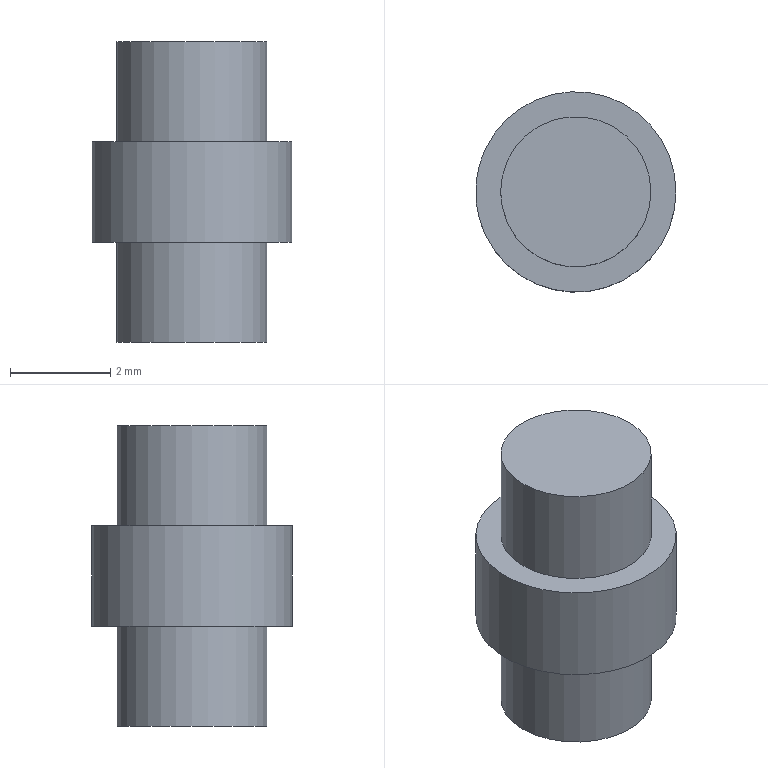Component | NX | CIRCUIT_PIN_2 | 1 solid | 7 faces | box 4 x 4 x 6 mm | volume 53 mm3 | plane 4 | cylinder 3 | commonest cylinder face diameters 3 x2 4 x1
STEP:
#1=CARTESIAN_POINT('',(0.,0.,0.));
#2=DIRECTION('',(0.,0.,1.));
#3=DIRECTION('',(1.,0.,0.));
#4=AXIS2_PLACEMENT_3D('',#1,#2,#3);
#5=CARTESIAN_POINT('',(22.205,25.006,-22.892));
#6=VERTEX_POINT('',#5);
#7=CARTESIAN_POINT('',(20.705,25.006,-22.892));
#8=DIRECTION('',(0.,0.,-1.));
#9=DIRECTION('',(1.,0.,0.));
#10=AXIS2_PLACEMENT_3D('',#7,#8,#9);
#11=CIRCLE('',#10,1.5);
#12=CARTESIAN_POINT('',(20.705,25.006,-22.892));
#13=DIRECTION('',(0.,0.,1.));
#14=DIRECTION('',(0.,-1.,0.));
#15=AXIS2_PLACEMENT_3D('',#12,#13,#14);
#16=PLANE('',#15);
#17=CARTESIAN_POINT('',(0.,1.5));
#18=CARTESIAN_POINT('',(2.598,1.5));
#19=CARTESIAN_POINT('',(1.299,-0.75));
#20=CARTESIAN_POINT('',(0.,-3.));
#21=CARTESIAN_POINT('',(-1.299,-0.75));
#22=CARTESIAN_POINT('',(-2.598,1.5));
#23=CARTESIAN_POINT('',(0.,1.5));
#24=(BOUNDED_CURVE()B_SPLINE_CURVE(2,(#17,#18,#19,#20,#21,#22,#23),.UNSPECIFIED.,.T.,.F.)B_SPLINE_CURVE_WITH_KNOTS((1,2,2,2,2,1),(-2.094,0.,2.094,4.189,6.283,8.378),.UNSPECIFIED.)CURVE()GEOMETRIC_REPRESENTATION_ITEM()RATIONAL_B_SPLINE_CURVE((1.,0.5,1.,0.5,1.,0.5,1.))REPRESENTATION_ITEM(''));
#25=(GEOMETRIC_REPRESENTATION_CONTEXT(2)PARAMETRIC_REPRESENTATION_CONTEXT()REPRESENTATION_CONTEXT('',''));
#26=DEFINITIONAL_REPRESENTATION('',(#24),#25);
#27=PCURVE('',#16,#26);
#28=CARTESIAN_POINT('',(20.705,25.006,-24.892));
#29=DIRECTION('',(0.,0.,1.));
#30=DIRECTION('',(1.,0.,0.));
#31=AXIS2_PLACEMENT_3D('',#28,#29,#30);
#32=CYLINDRICAL_SURFACE('',#31,1.5);
#33=CARTESIAN_POINT('',(6.283,2.));
#34=DIRECTION('',(-1.,0.));
#35=VECTOR('',#34,1.);
#36=LINE('',#33,#35);
#37=(GEOMETRIC_REPRESENTATION_CONTEXT(2)PARAMETRIC_REPRESENTATION_CONTEXT()REPRESENTATION_CONTEXT('',''));
#38=DEFINITIONAL_REPRESENTATION('',(#36),#37);
#39=PCURVE('',#32,#38);
#40=SURFACE_CURVE('',#11,(#27,#39),.PCURVE_S1.);
#41=EDGE_CURVE('',#6,#6,#40,.T.);
#42=ORIENTED_EDGE('',*,*,#41,.F.);
#43=EDGE_LOOP('',(#42));
#44=FACE_BOUND('',#43,.T.);
#45=ADVANCED_FACE('',(#44),#16,.T.);
#46=ORIENTED_EDGE('',*,*,#41,.T.);
#47=CARTESIAN_POINT('',(22.205,25.006,-24.892));
#48=VERTEX_POINT('',#47);
#49=CARTESIAN_POINT('',(22.205,25.006,-24.892));
#50=CARTESIAN_POINT('',(22.205,25.006,-22.892));
#51=B_SPLINE_CURVE_WITH_KNOTS('',1,(#49,#50),.UNSPECIFIED.,.F.,.F.,(2,2),(0.,2.),.PIECEWISE_BEZIER_KNOTS.);
#52=CARTESIAN_POINT('',(0.,0.));
#53=DIRECTION('',(0.,1.));
#54=VECTOR('',#53,1.);
#55=LINE('',#52,#54);
#56=(GEOMETRIC_REPRESENTATION_CONTEXT(2)PARAMETRIC_REPRESENTATION_CONTEXT()REPRESENTATION_CONTEXT('',''));
#57=DEFINITIONAL_REPRESENTATION('',(#55),#56);
#58=PCURVE('',#32,#57);
#59=CARTESIAN_POINT('',(6.283,0.));
#60=DIRECTION('',(0.,1.));
#61=VECTOR('',#60,1.);
#62=LINE('',#59,#61);
#63=(GEOMETRIC_REPRESENTATION_CONTEXT(2)PARAMETRIC_REPRESENTATION_CONTEXT()REPRESENTATION_CONTEXT('',''));
#64=DEFINITIONAL_REPRESENTATION('',(#62),#63);
#65=PCURVE('',#32,#64);
#66=SEAM_CURVE('',#51,(#58,#65),.PCURVE_S1.);
#67=EDGE_CURVE('',#48,#6,#66,.T.);
#68=ORIENTED_EDGE('',*,*,#67,.F.);
#69=CARTESIAN_POINT('',(20.705,25.006,-24.892));
#70=DIRECTION('',(0.,0.,1.));
#71=DIRECTION('',(1.,0.,0.));
#72=AXIS2_PLACEMENT_3D('',#69,#70,#71);
#73=CIRCLE('',#72,1.5);
#74=CARTESIAN_POINT('',(0.,0.));
#75=DIRECTION('',(1.,0.));
#76=VECTOR('',#75,1.);
#77=LINE('',#74,#76);
#78=(GEOMETRIC_REPRESENTATION_CONTEXT(2)PARAMETRIC_REPRESENTATION_CONTEXT()REPRESENTATION_CONTEXT('',''));
#79=DEFINITIONAL_REPRESENTATION('',(#77),#78);
#80=PCURVE('',#32,#79);
#81=CARTESIAN_POINT('',(20.705,25.006,-24.892));
#82=DIRECTION('',(0.,0.,1.));
#83=DIRECTION('',(0.,-1.,0.));
#84=AXIS2_PLACEMENT_3D('',#81,#82,#83);
#85=PLANE('',#84);
#86=CARTESIAN_POINT('',(0.,0.));
#87=DIRECTION('',(0.,1.));
#88=AXIS2_PLACEMENT_2D('',#86,#87);
#89=CIRCLE('',#88,1.5);
#90=(GEOMETRIC_REPRESENTATION_CONTEXT(2)PARAMETRIC_REPRESENTATION_CONTEXT()REPRESENTATION_CONTEXT('',''));
#91=DEFINITIONAL_REPRESENTATION('',(#89),#90);
#92=PCURVE('',#85,#91);
#93=SURFACE_CURVE('',#73,(#80,#92),.PCURVE_S1.);
#94=EDGE_CURVE('',#48,#48,#93,.T.);
#95=ORIENTED_EDGE('',*,*,#94,.T.);
#96=ORIENTED_EDGE('',*,*,#67,.T.);
#97=EDGE_LOOP('',(#46,#68,#95,#96));
#98=FACE_BOUND('',#97,.T.);
#99=ADVANCED_FACE('',(#98),#32,.T.);
#100=CARTESIAN_POINT('',(22.205,25.006,-26.892));
#101=VERTEX_POINT('',#100);
#102=CARTESIAN_POINT('',(20.705,25.006,-26.892));
#103=DIRECTION('',(0.,0.,-1.));
#104=DIRECTION('',(1.,0.,0.));
#105=AXIS2_PLACEMENT_3D('',#102,#103,#104);
#106=CIRCLE('',#105,1.5);
#107=CARTESIAN_POINT('',(20.705,25.006,-26.892));
#108=DIRECTION('',(0.,0.,-1.));
#109=DIRECTION('',(0.,1.,0.));
#110=AXIS2_PLACEMENT_3D('',#107,#108,#109);
#111=PLANE('',#110);
#112=CARTESIAN_POINT('',(0.,0.));
#113=DIRECTION('',(0.,1.));
#114=AXIS2_PLACEMENT_2D('',#112,#113);
#115=CIRCLE('',#114,1.5);
#116=(GEOMETRIC_REPRESENTATION_CONTEXT(2)PARAMETRIC_REPRESENTATION_CONTEXT()REPRESENTATION_CONTEXT('',''));
#117=DEFINITIONAL_REPRESENTATION('',(#115),#116);
#118=PCURVE('',#111,#117);
#119=CARTESIAN_POINT('',(20.705,25.006,-26.892));
#120=DIRECTION('',(0.,0.,-1.));
#121=DIRECTION('',(1.,0.,0.));
#122=AXIS2_PLACEMENT_3D('',#119,#120,#121);
#123=CYLINDRICAL_SURFACE('',#122,1.5);
#124=CARTESIAN_POINT('',(0.,0.));
#125=DIRECTION('',(1.,0.));
#126=VECTOR('',#125,1.);
#127=LINE('',#124,#126);
#128=(GEOMETRIC_REPRESENTATION_CONTEXT(2)PARAMETRIC_REPRESENTATION_CONTEXT()REPRESENTATION_CONTEXT('',''));
#129=DEFINITIONAL_REPRESENTATION('',(#127),#128);
#130=PCURVE('',#123,#129);
#131=SURFACE_CURVE('',#106,(#118,#130),.PCURVE_S1.);
#132=EDGE_CURVE('',#101,#101,#131,.T.);
#133=ORIENTED_EDGE('',*,*,#132,.F.);
#134=EDGE_LOOP('',(#133));
#135=FACE_BOUND('',#134,.T.);
#136=CARTESIAN_POINT('',(22.705,25.006,-26.892));
#137=VERTEX_POINT('',#136);
#138=CARTESIAN_POINT('',(20.705,25.006,-26.892));
#139=DIRECTION('',(0.,0.,1.));
#140=DIRECTION('',(1.,0.,0.));
#141=AXIS2_PLACEMENT_3D('',#138,#139,#140);
#142=CIRCLE('',#141,2.);
#143=CARTESIAN_POINT('',(0.,2.));
#144=CARTESIAN_POINT('',(3.464,2.));
#145=CARTESIAN_POINT('',(1.732,-1.));
#146=CARTESIAN_POINT('',(0.,-4.));
#147=CARTESIAN_POINT('',(-1.732,-1.));
#148=CARTESIAN_POINT('',(-3.464,2.));
#149=CARTESIAN_POINT('',(0.,2.));
#150=(BOUNDED_CURVE()B_SPLINE_CURVE(2,(#143,#144,#145,#146,#147,#148,#149),.UNSPECIFIED.,.T.,.F.)B_SPLINE_CURVE_WITH_KNOTS((1,2,2,2,2,1),(-2.094,0.,2.094,4.189,6.283,8.378),.UNSPECIFIED.)CURVE()GEOMETRIC_REPRESENTATION_ITEM()RATIONAL_B_SPLINE_CURVE((1.,0.5,1.,0.5,1.,0.5,1.))REPRESENTATION_ITEM(''));
#151=(GEOMETRIC_REPRESENTATION_CONTEXT(2)PARAMETRIC_REPRESENTATION_CONTEXT()REPRESENTATION_CONTEXT('',''));
#152=DEFINITIONAL_REPRESENTATION('',(#150),#151);
#153=PCURVE('',#111,#152);
#154=CARTESIAN_POINT('',(20.705,25.006,-24.892));
#155=DIRECTION('',(0.,0.,-1.));
#156=DIRECTION('',(1.,0.,0.));
#157=AXIS2_PLACEMENT_3D('',#154,#155,#156);
#158=CYLINDRICAL_SURFACE('',#157,2.);
#159=CARTESIAN_POINT('',(6.283,2.));
#160=DIRECTION('',(-1.,0.));
#161=VECTOR('',#160,1.);
#162=LINE('',#159,#161);
#163=(GEOMETRIC_REPRESENTATION_CONTEXT(2)PARAMETRIC_REPRESENTATION_CONTEXT()REPRESENTATION_CONTEXT('',''));
#164=DEFINITIONAL_REPRESENTATION('',(#162),#163);
#165=PCURVE('',#158,#164);
#166=SURFACE_CURVE('',#142,(#153,#165),.PCURVE_S1.);
#167=EDGE_CURVE('',#137,#137,#166,.T.);
#168=ORIENTED_EDGE('',*,*,#167,.F.);
#169=EDGE_LOOP('',(#168));
#170=FACE_BOUND('',#169,.T.);
#171=ADVANCED_FACE('',(#135,#170),#111,.T.);
#172=ORIENTED_EDGE('',*,*,#94,.F.);
#173=EDGE_LOOP('',(#172));
#174=FACE_BOUND('',#173,.T.);
#175=CARTESIAN_POINT('',(22.705,25.006,-24.892));
#176=VERTEX_POINT('',#175);
#177=CARTESIAN_POINT('',(20.705,25.006,-24.892));
#178=DIRECTION('',(0.,0.,-1.));
#179=DIRECTION('',(1.,0.,0.));
#180=AXIS2_PLACEMENT_3D('',#177,#178,#179);
#181=CIRCLE('',#180,2.);
#182=CARTESIAN_POINT('',(0.,2.));
#183=CARTESIAN_POINT('',(3.464,2.));
#184=CARTESIAN_POINT('',(1.732,-1.));
#185=CARTESIAN_POINT('',(0.,-4.));
#186=CARTESIAN_POINT('',(-1.732,-1.));
#187=CARTESIAN_POINT('',(-3.464,2.));
#188=CARTESIAN_POINT('',(0.,2.));
#189=(BOUNDED_CURVE()B_SPLINE_CURVE(2,(#182,#183,#184,#185,#186,#187,#188),.UNSPECIFIED.,.T.,.F.)B_SPLINE_CURVE_WITH_KNOTS((1,2,2,2,2,1),(-2.094,0.,2.094,4.189,6.283,8.378),.UNSPECIFIED.)CURVE()GEOMETRIC_REPRESENTATION_ITEM()RATIONAL_B_SPLINE_CURVE((1.,0.5,1.,0.5,1.,0.5,1.))REPRESENTATION_ITEM(''));
#190=(GEOMETRIC_REPRESENTATION_CONTEXT(2)PARAMETRIC_REPRESENTATION_CONTEXT()REPRESENTATION_CONTEXT('',''));
#191=DEFINITIONAL_REPRESENTATION('',(#189),#190);
#192=PCURVE('',#85,#191);
#193=CARTESIAN_POINT('',(0.,0.));
#194=DIRECTION('',(1.,0.));
#195=VECTOR('',#194,1.);
#196=LINE('',#193,#195);
#197=(GEOMETRIC_REPRESENTATION_CONTEXT(2)PARAMETRIC_REPRESENTATION_CONTEXT()REPRESENTATION_CONTEXT('',''));
#198=DEFINITIONAL_REPRESENTATION('',(#196),#197);
#199=PCURVE('',#158,#198);
#200=SURFACE_CURVE('',#181,(#192,#199),.PCURVE_S1.);
#201=EDGE_CURVE('',#176,#176,#200,.T.);
#202=ORIENTED_EDGE('',*,*,#201,.F.);
#203=EDGE_LOOP('',(#202));
#204=FACE_BOUND('',#203,.T.);
#205=ADVANCED_FACE('',(#174,#204),#85,.T.);
#206=ORIENTED_EDGE('',*,*,#167,.T.);
#207=CARTESIAN_POINT('',(22.705,25.006,-24.892));
#208=CARTESIAN_POINT('',(22.705,25.006,-26.892));
#209=B_SPLINE_CURVE_WITH_KNOTS('',1,(#207,#208),.UNSPECIFIED.,.F.,.F.,(2,2),(0.,2.),.PIECEWISE_BEZIER_KNOTS.);
#210=CARTESIAN_POINT('',(0.,0.));
#211=DIRECTION('',(0.,1.));
#212=VECTOR('',#211,1.);
#213=LINE('',#210,#212);
#214=(GEOMETRIC_REPRESENTATION_CONTEXT(2)PARAMETRIC_REPRESENTATION_CONTEXT()REPRESENTATION_CONTEXT('',''));
#215=DEFINITIONAL_REPRESENTATION('',(#213),#214);
#216=PCURVE('',#158,#215);
#217=CARTESIAN_POINT('',(6.283,0.));
#218=DIRECTION('',(0.,1.));
#219=VECTOR('',#218,1.);
#220=LINE('',#217,#219);
#221=(GEOMETRIC_REPRESENTATION_CONTEXT(2)PARAMETRIC_REPRESENTATION_CONTEXT()REPRESENTATION_CONTEXT('',''));
#222=DEFINITIONAL_REPRESENTATION('',(#220),#221);
#223=PCURVE('',#158,#222);
#224=SEAM_CURVE('',#209,(#216,#223),.PCURVE_S1.);
#225=EDGE_CURVE('',#176,#137,#224,.T.);
#226=ORIENTED_EDGE('',*,*,#225,.F.);
#227=ORIENTED_EDGE('',*,*,#201,.T.);
#228=ORIENTED_EDGE('',*,*,#225,.T.);
#229=EDGE_LOOP('',(#206,#226,#227,#228));
#230=FACE_BOUND('',#229,.T.);
#231=ADVANCED_FACE('',(#230),#158,.T.);
#232=CARTESIAN_POINT('',(22.205,25.006,-28.892));
#233=VERTEX_POINT('',#232);
#234=CARTESIAN_POINT('',(20.705,25.006,-28.892));
#235=DIRECTION('',(0.,0.,1.));
#236=DIRECTION('',(1.,0.,0.));
#237=AXIS2_PLACEMENT_3D('',#234,#235,#236);
#238=CIRCLE('',#237,1.5);
#239=CARTESIAN_POINT('',(20.705,25.006,-28.892));
#240=DIRECTION('',(0.,0.,-1.));
#241=DIRECTION('',(0.,1.,0.));
#242=AXIS2_PLACEMENT_3D('',#239,#240,#241);
#243=PLANE('',#242);
#244=CARTESIAN_POINT('',(0.,1.5));
#245=CARTESIAN_POINT('',(2.598,1.5));
#246=CARTESIAN_POINT('',(1.299,-0.75));
#247=CARTESIAN_POINT('',(0.,-3.));
#248=CARTESIAN_POINT('',(-1.299,-0.75));
#249=CARTESIAN_POINT('',(-2.598,1.5));
#250=CARTESIAN_POINT('',(0.,1.5));
#251=(BOUNDED_CURVE()B_SPLINE_CURVE(2,(#244,#245,#246,#247,#248,#249,#250),.UNSPECIFIED.,.T.,.F.)B_SPLINE_CURVE_WITH_KNOTS((1,2,2,2,2,1),(-2.094,0.,2.094,4.189,6.283,8.378),.UNSPECIFIED.)CURVE()GEOMETRIC_REPRESENTATION_ITEM()RATIONAL_B_SPLINE_CURVE((1.,0.5,1.,0.5,1.,0.5,1.))REPRESENTATION_ITEM(''));
#252=(GEOMETRIC_REPRESENTATION_CONTEXT(2)PARAMETRIC_REPRESENTATION_CONTEXT()REPRESENTATION_CONTEXT('',''));
#253=DEFINITIONAL_REPRESENTATION('',(#251),#252);
#254=PCURVE('',#243,#253);
#255=CARTESIAN_POINT('',(6.283,2.));
#256=DIRECTION('',(-1.,0.));
#257=VECTOR('',#256,1.);
#258=LINE('',#255,#257);
#259=(GEOMETRIC_REPRESENTATION_CONTEXT(2)PARAMETRIC_REPRESENTATION_CONTEXT()REPRESENTATION_CONTEXT('',''));
#260=DEFINITIONAL_REPRESENTATION('',(#258),#259);
#261=PCURVE('',#123,#260);
#262=SURFACE_CURVE('',#238,(#254,#261),.PCURVE_S1.);
#263=EDGE_CURVE('',#233,#233,#262,.T.);
#264=ORIENTED_EDGE('',*,*,#263,.F.);
#265=EDGE_LOOP('',(#264));
#266=FACE_BOUND('',#265,.T.);
#267=ADVANCED_FACE('',(#266),#243,.T.);
#268=ORIENTED_EDGE('',*,*,#263,.T.);
#269=CARTESIAN_POINT('',(22.205,25.006,-26.892));
#270=CARTESIAN_POINT('',(22.205,25.006,-28.892));
#271=B_SPLINE_CURVE_WITH_KNOTS('',1,(#269,#270),.UNSPECIFIED.,.F.,.F.,(2,2),(0.,2.),.PIECEWISE_BEZIER_KNOTS.);
#272=CARTESIAN_POINT('',(0.,0.));
#273=DIRECTION('',(0.,1.));
#274=VECTOR('',#273,1.);
#275=LINE('',#272,#274);
#276=(GEOMETRIC_REPRESENTATION_CONTEXT(2)PARAMETRIC_REPRESENTATION_CONTEXT()REPRESENTATION_CONTEXT('',''));
#277=DEFINITIONAL_REPRESENTATION('',(#275),#276);
#278=PCURVE('',#123,#277);
#279=CARTESIAN_POINT('',(6.283,0.));
#280=DIRECTION('',(0.,1.));
#281=VECTOR('',#280,1.);
#282=LINE('',#279,#281);
#283=(GEOMETRIC_REPRESENTATION_CONTEXT(2)PARAMETRIC_REPRESENTATION_CONTEXT()REPRESENTATION_CONTEXT('',''));
#284=DEFINITIONAL_REPRESENTATION('',(#282),#283);
#285=PCURVE('',#123,#284);
#286=SEAM_CURVE('',#271,(#278,#285),.PCURVE_S1.);
#287=EDGE_CURVE('',#101,#233,#286,.T.);
#288=ORIENTED_EDGE('',*,*,#287,.F.);
#289=ORIENTED_EDGE('',*,*,#132,.T.);
#290=ORIENTED_EDGE('',*,*,#287,.T.);
#291=EDGE_LOOP('',(#268,#288,#289,#290));
#292=FACE_BOUND('',#291,.T.);
#293=ADVANCED_FACE('',(#292),#123,.T.);
#294=CLOSED_SHELL('',(#45,#99,#171,#205,#231,#267,#293));
#295=MANIFOLD_SOLID_BREP('',#294);
#296=(LENGTH_UNIT()NAMED_UNIT(*)SI_UNIT(.MILLI.,.METRE.));
#297=UNCERTAINTY_MEASURE_WITH_UNIT(LENGTH_MEASURE(0.00001),#296,'','');
#298=(NAMED_UNIT(*)PLANE_ANGLE_UNIT()SI_UNIT($,.RADIAN.));
#299=(NAMED_UNIT(*)SI_UNIT($,.STERADIAN.)SOLID_ANGLE_UNIT());
#300=(GEOMETRIC_REPRESENTATION_CONTEXT(3)GLOBAL_UNCERTAINTY_ASSIGNED_CONTEXT((#297))GLOBAL_UNIT_ASSIGNED_CONTEXT((#296,#298,#299))REPRESENTATION_CONTEXT('',''));
#301=ADVANCED_BREP_SHAPE_REPRESENTATION('',(#4,#295),#300);